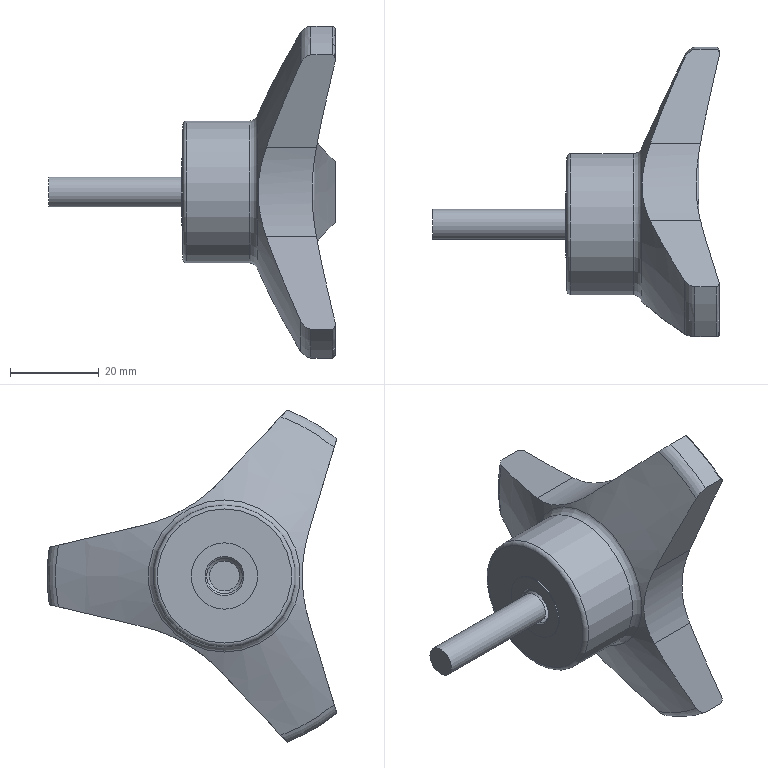Component | NX | 65672_X_T | 2 solids | 36 faces | volume 39002 mm3 | plane 12 | cylinder 11 | torus 9 | cone 4 | commonest cylinder face diameters 80 x3 70 x3 8 x1 21 x1 32 x1 15 x1 6.8 x1